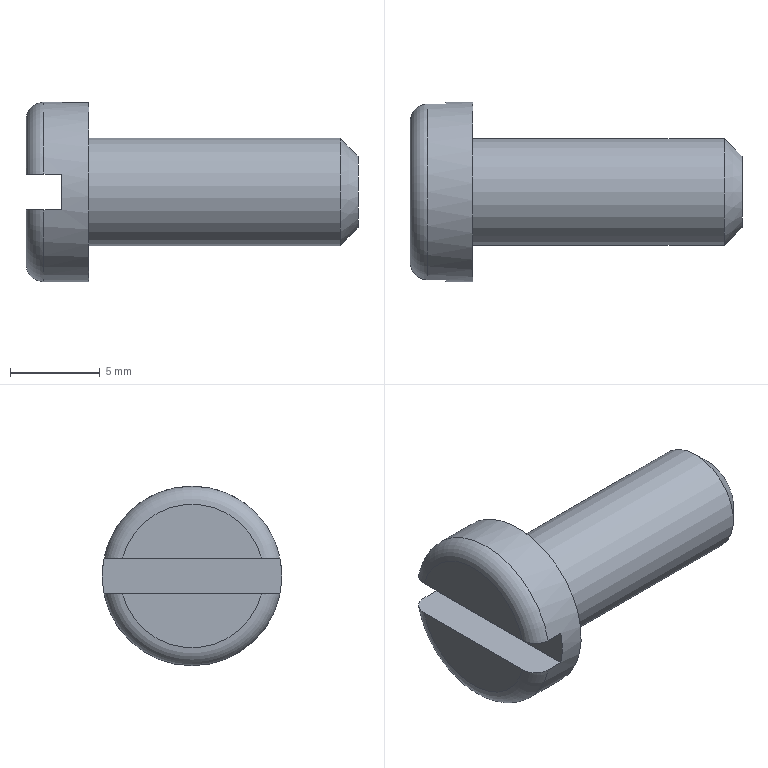Component | NX | SLOTTED_CAP_SCREW | 1 solid | 12 faces | box 18.5 x 10 x 10 mm | volume 645 mm3 | plane 7 | cylinder 2 | torus 2 | cone 1 | commonest cylinder face diameters 10 x1 6 x1
STEP:
#1=CARTESIAN_POINT('',(0.,0.,0.));
#2=DIRECTION('',(0.,0.,1.));
#3=DIRECTION('',(1.,0.,0.));
#4=AXIS2_PLACEMENT_3D('',#1,#2,#3);
#5=CARTESIAN_POINT('',(-33.6,-11.127,-0.5));
#6=VERTEX_POINT('',#5);
#7=CARTESIAN_POINT('',(-33.6,-18.873,-0.5));
#8=VERTEX_POINT('',#7);
#9=CARTESIAN_POINT('',(-33.6,11.305,-0.5));
#10=DIRECTION('',(0.,-1.,0.));
#11=VECTOR('',#10,1.);
#12=LINE('',#9,#11);
#13=CARTESIAN_POINT('',(-33.6,-15.,0.5));
#14=DIRECTION('',(-1.,0.,0.));
#15=DIRECTION('',(0.,0.,-1.));
#16=AXIS2_PLACEMENT_3D('',#13,#14,#15);
#17=PLANE('',#16);
#18=CARTESIAN_POINT('',(1.,-26.305));
#19=DIRECTION('',(0.,1.));
#20=VECTOR('',#19,1.);
#21=LINE('',#18,#20);
#22=(GEOMETRIC_REPRESENTATION_CONTEXT(2)PARAMETRIC_REPRESENTATION_CONTEXT()REPRESENTATION_CONTEXT('',''));
#23=DEFINITIONAL_REPRESENTATION('',(#21),#22);
#24=PCURVE('',#17,#23);
#25=CARTESIAN_POINT('',(-33.6,11.305,-0.5));
#26=DIRECTION('',(0.,0.,-1.));
#27=DIRECTION('',(1.,0.,0.));
#28=AXIS2_PLACEMENT_3D('',#25,#26,#27);
#29=PLANE('',#28);
#30=CARTESIAN_POINT('',(0.,0.));
#31=DIRECTION('',(0.,1.));
#32=VECTOR('',#31,1.);
#33=LINE('',#30,#32);
#34=(GEOMETRIC_REPRESENTATION_CONTEXT(2)PARAMETRIC_REPRESENTATION_CONTEXT()REPRESENTATION_CONTEXT('',''));
#35=DEFINITIONAL_REPRESENTATION('',(#33),#34);
#36=PCURVE('',#29,#35);
#37=SURFACE_CURVE('',#12,(#24,#36),.PCURVE_S1.);
#38=EDGE_CURVE('',#6,#8,#37,.T.);
#39=ORIENTED_EDGE('',*,*,#38,.F.);
#40=CARTESIAN_POINT('',(-33.6,-15.,0.5));
#41=DIRECTION('',(-1.,0.,0.));
#42=DIRECTION('',(0.,0.,-1.));
#43=AXIS2_PLACEMENT_3D('',#40,#41,#42);
#44=CIRCLE('',#43,4.);
#45=CARTESIAN_POINT('',(0.,0.));
#46=DIRECTION('',(1.,0.));
#47=AXIS2_PLACEMENT_2D('',#45,#46);
#48=CIRCLE('',#47,4.);
#49=(GEOMETRIC_REPRESENTATION_CONTEXT(2)PARAMETRIC_REPRESENTATION_CONTEXT()REPRESENTATION_CONTEXT('',''));
#50=DEFINITIONAL_REPRESENTATION('',(#48),#49);
#51=PCURVE('',#17,#50);
#52=CARTESIAN_POINT('',(-32.6,-15.,0.5));
#53=DIRECTION('',(-1.,0.,0.));
#54=DIRECTION('',(0.,0.,-1.));
#55=AXIS2_PLACEMENT_3D('',#52,#53,#54);
#56=TOROIDAL_SURFACE('',#55,4.,1.);
#57=CARTESIAN_POINT('',(0.,1.571));
#58=DIRECTION('',(1.,-0.));
#59=VECTOR('',#58,1.);
#60=LINE('',#57,#59);
#61=(GEOMETRIC_REPRESENTATION_CONTEXT(2)PARAMETRIC_REPRESENTATION_CONTEXT()REPRESENTATION_CONTEXT('',''));
#62=DEFINITIONAL_REPRESENTATION('',(#60),#61);
#63=PCURVE('',#56,#62);
#64=SURFACE_CURVE('',#44,(#51,#63),.PCURVE_S1.);
#65=EDGE_CURVE('',#6,#8,#64,.T.);
#66=ORIENTED_EDGE('',*,*,#65,.T.);
#67=EDGE_LOOP('',(#39,#66));
#68=FACE_BOUND('',#67,.T.);
#69=ADVANCED_FACE('',(#68),#17,.T.);
#70=CARTESIAN_POINT('',(-33.6,-11.127,1.5));
#71=VERTEX_POINT('',#70);
#72=CARTESIAN_POINT('',(-33.6,-18.873,1.5));
#73=VERTEX_POINT('',#72);
#74=CARTESIAN_POINT('',(-33.6,11.305,1.5));
#75=DIRECTION('',(0.,-1.,0.));
#76=VECTOR('',#75,1.);
#77=LINE('',#74,#76);
#78=CARTESIAN_POINT('',(-33.6,-15.,0.5));
#79=DIRECTION('',(-1.,0.,0.));
#80=DIRECTION('',(0.,0.,-1.));
#81=AXIS2_PLACEMENT_3D('',#78,#79,#80);
#82=PLANE('',#81);
#83=CARTESIAN_POINT('',(-1.,-26.305));
#84=DIRECTION('',(0.,1.));
#85=VECTOR('',#84,1.);
#86=LINE('',#83,#85);
#87=(GEOMETRIC_REPRESENTATION_CONTEXT(2)PARAMETRIC_REPRESENTATION_CONTEXT()REPRESENTATION_CONTEXT('',''));
#88=DEFINITIONAL_REPRESENTATION('',(#86),#87);
#89=PCURVE('',#82,#88);
#90=CARTESIAN_POINT('',(-33.6,-38.695,1.5));
#91=DIRECTION('',(0.,0.,1.));
#92=DIRECTION('',(-1.,0.,0.));
#93=AXIS2_PLACEMENT_3D('',#90,#91,#92);
#94=PLANE('',#93);
#95=CARTESIAN_POINT('',(0.,-50.));
#96=DIRECTION('',(0.,1.));
#97=VECTOR('',#96,1.);
#98=LINE('',#95,#97);
#99=(GEOMETRIC_REPRESENTATION_CONTEXT(2)PARAMETRIC_REPRESENTATION_CONTEXT()REPRESENTATION_CONTEXT('',''));
#100=DEFINITIONAL_REPRESENTATION('',(#98),#99);
#101=PCURVE('',#94,#100);
#102=SURFACE_CURVE('',#77,(#89,#101),.PCURVE_S1.);
#103=EDGE_CURVE('',#71,#73,#102,.T.);
#104=ORIENTED_EDGE('',*,*,#103,.T.);
#105=CARTESIAN_POINT('',(-33.6,-15.,0.5));
#106=DIRECTION('',(-1.,0.,0.));
#107=DIRECTION('',(0.,0.,-1.));
#108=AXIS2_PLACEMENT_3D('',#105,#106,#107);
#109=CIRCLE('',#108,4.);
#110=CARTESIAN_POINT('',(0.,0.));
#111=DIRECTION('',(1.,0.));
#112=AXIS2_PLACEMENT_2D('',#110,#111);
#113=CIRCLE('',#112,4.);
#114=(GEOMETRIC_REPRESENTATION_CONTEXT(2)PARAMETRIC_REPRESENTATION_CONTEXT()REPRESENTATION_CONTEXT('',''));
#115=DEFINITIONAL_REPRESENTATION('',(#113),#114);
#116=PCURVE('',#82,#115);
#117=CARTESIAN_POINT('',(-32.6,-15.,0.5));
#118=DIRECTION('',(-1.,0.,0.));
#119=DIRECTION('',(0.,0.,-1.));
#120=AXIS2_PLACEMENT_3D('',#117,#118,#119);
#121=TOROIDAL_SURFACE('',#120,4.,1.);
#122=CARTESIAN_POINT('',(0.,1.571));
#123=DIRECTION('',(1.,-0.));
#124=VECTOR('',#123,1.);
#125=LINE('',#122,#124);
#126=(GEOMETRIC_REPRESENTATION_CONTEXT(2)PARAMETRIC_REPRESENTATION_CONTEXT()REPRESENTATION_CONTEXT('',''));
#127=DEFINITIONAL_REPRESENTATION('',(#125),#126);
#128=PCURVE('',#121,#127);
#129=SURFACE_CURVE('',#109,(#116,#128),.PCURVE_S1.);
#130=EDGE_CURVE('',#73,#71,#129,.T.);
#131=ORIENTED_EDGE('',*,*,#130,.T.);
#132=EDGE_LOOP('',(#104,#131));
#133=FACE_BOUND('',#132,.T.);
#134=ADVANCED_FACE('',(#133),#82,.T.);
#135=CARTESIAN_POINT('',(-30.1,-15.,3.5));
#136=VERTEX_POINT('',#135);
#137=CARTESIAN_POINT('',(-30.1,-15.,0.5));
#138=DIRECTION('',(1.,0.,0.));
#139=DIRECTION('',(0.,0.,1.));
#140=AXIS2_PLACEMENT_3D('',#137,#138,#139);
#141=CIRCLE('',#140,3.);
#142=CARTESIAN_POINT('',(-30.1,-15.,0.5));
#143=DIRECTION('',(1.,0.,0.));
#144=DIRECTION('',(0.,0.,1.));
#145=AXIS2_PLACEMENT_3D('',#142,#143,#144);
#146=PLANE('',#145);
#147=CARTESIAN_POINT('',(-0.,0.));
#148=DIRECTION('',(1.,0.));
#149=AXIS2_PLACEMENT_2D('',#147,#148);
#150=CIRCLE('',#149,3.);
#151=(GEOMETRIC_REPRESENTATION_CONTEXT(2)PARAMETRIC_REPRESENTATION_CONTEXT()REPRESENTATION_CONTEXT('',''));
#152=DEFINITIONAL_REPRESENTATION('',(#150),#151);
#153=PCURVE('',#146,#152);
#154=CARTESIAN_POINT('',(-30.1,-15.,0.5));
#155=DIRECTION('',(1.,0.,0.));
#156=DIRECTION('',(0.,0.,1.));
#157=AXIS2_PLACEMENT_3D('',#154,#155,#156);
#158=CYLINDRICAL_SURFACE('',#157,3.);
#159=CARTESIAN_POINT('',(0.,0.));
#160=DIRECTION('',(1.,0.));
#161=VECTOR('',#160,1.);
#162=LINE('',#159,#161);
#163=(GEOMETRIC_REPRESENTATION_CONTEXT(2)PARAMETRIC_REPRESENTATION_CONTEXT()REPRESENTATION_CONTEXT('',''));
#164=DEFINITIONAL_REPRESENTATION('',(#162),#163);
#165=PCURVE('',#158,#164);
#166=SURFACE_CURVE('',#141,(#153,#165),.PCURVE_S1.);
#167=EDGE_CURVE('',#136,#136,#166,.T.);
#168=ORIENTED_EDGE('',*,*,#167,.F.);
#169=EDGE_LOOP('',(#168));
#170=FACE_BOUND('',#169,.T.);
#171=CARTESIAN_POINT('',(-30.1,-15.,-4.5));
#172=VERTEX_POINT('',#171);
#173=CARTESIAN_POINT('',(-30.1,-15.,0.5));
#174=DIRECTION('',(-1.,0.,0.));
#175=DIRECTION('',(0.,0.,-1.));
#176=AXIS2_PLACEMENT_3D('',#173,#174,#175);
#177=CIRCLE('',#176,5.);
#178=CARTESIAN_POINT('',(-5.,0.));
#179=CARTESIAN_POINT('',(-5.,8.66));
#180=CARTESIAN_POINT('',(2.5,4.33));
#181=CARTESIAN_POINT('',(10.,0.));
#182=CARTESIAN_POINT('',(2.5,-4.33));
#183=CARTESIAN_POINT('',(-5.,-8.66));
#184=CARTESIAN_POINT('',(-5.,0.));
#185=(BOUNDED_CURVE()B_SPLINE_CURVE(2,(#178,#179,#180,#181,#182,#183,#184),.UNSPECIFIED.,.T.,.F.)B_SPLINE_CURVE_WITH_KNOTS((1,2,2,2,2,1),(-2.094,0.,2.094,4.189,6.283,8.378),.UNSPECIFIED.)CURVE()GEOMETRIC_REPRESENTATION_ITEM()RATIONAL_B_SPLINE_CURVE((1.,0.5,1.,0.5,1.,0.5,1.))REPRESENTATION_ITEM(''));
#186=(GEOMETRIC_REPRESENTATION_CONTEXT(2)PARAMETRIC_REPRESENTATION_CONTEXT()REPRESENTATION_CONTEXT('',''));
#187=DEFINITIONAL_REPRESENTATION('',(#185),#186);
#188=PCURVE('',#146,#187);
#189=CARTESIAN_POINT('',(-30.1,-15.,0.5));
#190=DIRECTION('',(-1.,0.,0.));
#191=DIRECTION('',(0.,0.,-1.));
#192=AXIS2_PLACEMENT_3D('',#189,#190,#191);
#193=CYLINDRICAL_SURFACE('',#192,5.);
#194=CARTESIAN_POINT('',(0.,0.));
#195=DIRECTION('',(1.,0.));
#196=VECTOR('',#195,1.);
#197=LINE('',#194,#196);
#198=(GEOMETRIC_REPRESENTATION_CONTEXT(2)PARAMETRIC_REPRESENTATION_CONTEXT()REPRESENTATION_CONTEXT('',''));
#199=DEFINITIONAL_REPRESENTATION('',(#197),#198);
#200=PCURVE('',#193,#199);
#201=SURFACE_CURVE('',#177,(#188,#200),.PCURVE_S1.);
#202=EDGE_CURVE('',#172,#172,#201,.T.);
#203=ORIENTED_EDGE('',*,*,#202,.F.);
#204=EDGE_LOOP('',(#203));
#205=FACE_BOUND('',#204,.T.);
#206=ADVANCED_FACE('',(#170,#205),#146,.T.);
#207=CARTESIAN_POINT('',(-32.6,-19.899,-0.5));
#208=VERTEX_POINT('',#207);
#209=CARTESIAN_POINT('',(-31.6,-19.899,-0.5));
#210=VERTEX_POINT('',#209);
#211=CARTESIAN_POINT('',(-30.1,-19.899,-0.5));
#212=DIRECTION('',(1.,0.,0.));
#213=VECTOR('',#212,1.);
#214=LINE('',#211,#213);
#215=CARTESIAN_POINT('',(1.369,0.));
#216=DIRECTION('',(0.,-1.));
#217=VECTOR('',#216,1.);
#218=LINE('',#215,#217);
#219=(GEOMETRIC_REPRESENTATION_CONTEXT(2)PARAMETRIC_REPRESENTATION_CONTEXT()REPRESENTATION_CONTEXT('',''));
#220=DEFINITIONAL_REPRESENTATION('',(#218),#219);
#221=PCURVE('',#193,#220);
#222=CARTESIAN_POINT('',(3.5,31.204));
#223=DIRECTION('',(1.,0.));
#224=VECTOR('',#223,1.);
#225=LINE('',#222,#224);
#226=(GEOMETRIC_REPRESENTATION_CONTEXT(2)PARAMETRIC_REPRESENTATION_CONTEXT()REPRESENTATION_CONTEXT('',''));
#227=DEFINITIONAL_REPRESENTATION('',(#225),#226);
#228=PCURVE('',#29,#227);
#229=SURFACE_CURVE('',#214,(#221,#228),.PCURVE_S1.);
#230=EDGE_CURVE('',#208,#210,#229,.T.);
#231=ORIENTED_EDGE('',*,*,#230,.F.);
#232=CARTESIAN_POINT('',(-32.6,-15.,-4.5));
#233=VERTEX_POINT('',#232);
#234=CARTESIAN_POINT('',(-32.6,-15.,0.5));
#235=DIRECTION('',(1.,0.,0.));
#236=DIRECTION('',(0.,0.,-1.));
#237=AXIS2_PLACEMENT_3D('',#234,#235,#236);
#238=CIRCLE('',#237,5.);
#239=CARTESIAN_POINT('',(6.283,2.5));
#240=DIRECTION('',(-1.,0.));
#241=VECTOR('',#240,1.);
#242=LINE('',#239,#241);
#243=(GEOMETRIC_REPRESENTATION_CONTEXT(2)PARAMETRIC_REPRESENTATION_CONTEXT()REPRESENTATION_CONTEXT('',''));
#244=DEFINITIONAL_REPRESENTATION('',(#242),#243);
#245=PCURVE('',#193,#244);
#246=CARTESIAN_POINT('',(12.566,0.));
#247=DIRECTION('',(-1.,0.));
#248=VECTOR('',#247,1.);
#249=LINE('',#246,#248);
#250=(GEOMETRIC_REPRESENTATION_CONTEXT(2)PARAMETRIC_REPRESENTATION_CONTEXT()REPRESENTATION_CONTEXT('',''));
#251=DEFINITIONAL_REPRESENTATION('',(#249),#250);
#252=PCURVE('',#56,#251);
#253=SURFACE_CURVE('',#238,(#245,#252),.PCURVE_S1.);
#254=EDGE_CURVE('',#208,#233,#253,.T.);
#255=ORIENTED_EDGE('',*,*,#254,.T.);
#256=CARTESIAN_POINT('',(-30.1,-15.,-4.5));
#257=CARTESIAN_POINT('',(-32.6,-15.,-4.5));
#258=B_SPLINE_CURVE_WITH_KNOTS('',1,(#256,#257),.UNSPECIFIED.,.F.,.F.,(2,2),(0.,2.5),.PIECEWISE_BEZIER_KNOTS.);
#259=CARTESIAN_POINT('',(0.,0.));
#260=DIRECTION('',(0.,1.));
#261=VECTOR('',#260,1.);
#262=LINE('',#259,#261);
#263=(GEOMETRIC_REPRESENTATION_CONTEXT(2)PARAMETRIC_REPRESENTATION_CONTEXT()REPRESENTATION_CONTEXT('',''));
#264=DEFINITIONAL_REPRESENTATION('',(#262),#263);
#265=PCURVE('',#193,#264);
#266=CARTESIAN_POINT('',(6.283,0.));
#267=DIRECTION('',(0.,1.));
#268=VECTOR('',#267,1.);
#269=LINE('',#266,#268);
#270=(GEOMETRIC_REPRESENTATION_CONTEXT(2)PARAMETRIC_REPRESENTATION_CONTEXT()REPRESENTATION_CONTEXT('',''));
#271=DEFINITIONAL_REPRESENTATION('',(#269),#270);
#272=PCURVE('',#193,#271);
#273=SEAM_CURVE('',#258,(#265,#272),.PCURVE_S1.);
#274=EDGE_CURVE('',#172,#233,#273,.T.);
#275=ORIENTED_EDGE('',*,*,#274,.F.);
#276=ORIENTED_EDGE('',*,*,#202,.T.);
#277=ORIENTED_EDGE('',*,*,#274,.T.);
#278=CARTESIAN_POINT('',(-32.6,-10.101,-0.5));
#279=VERTEX_POINT('',#278);
#280=CARTESIAN_POINT('',(-32.6,-15.,0.5));
#281=DIRECTION('',(1.,0.,0.));
#282=DIRECTION('',(0.,0.,-1.));
#283=AXIS2_PLACEMENT_3D('',#280,#281,#282);
#284=CIRCLE('',#283,5.);
#285=CARTESIAN_POINT('',(12.566,2.5));
#286=DIRECTION('',(-1.,0.));
#287=VECTOR('',#286,1.);
#288=LINE('',#285,#287);
#289=(GEOMETRIC_REPRESENTATION_CONTEXT(2)PARAMETRIC_REPRESENTATION_CONTEXT()REPRESENTATION_CONTEXT('',''));
#290=DEFINITIONAL_REPRESENTATION('',(#288),#289);
#291=PCURVE('',#193,#290);
#292=CARTESIAN_POINT('',(12.566,0.));
#293=DIRECTION('',(-1.,0.));
#294=VECTOR('',#293,1.);
#295=LINE('',#292,#294);
#296=(GEOMETRIC_REPRESENTATION_CONTEXT(2)PARAMETRIC_REPRESENTATION_CONTEXT()REPRESENTATION_CONTEXT('',''));
#297=DEFINITIONAL_REPRESENTATION('',(#295),#296);
#298=PCURVE('',#56,#297);
#299=SURFACE_CURVE('',#284,(#291,#298),.PCURVE_S1.);
#300=EDGE_CURVE('',#233,#279,#299,.T.);
#301=ORIENTED_EDGE('',*,*,#300,.T.);
#302=CARTESIAN_POINT('',(-31.6,-10.101,-0.5));
#303=VERTEX_POINT('',#302);
#304=CARTESIAN_POINT('',(-30.1,-10.101,-0.5));
#305=DIRECTION('',(-1.,0.,0.));
#306=VECTOR('',#305,1.);
#307=LINE('',#304,#306);
#308=CARTESIAN_POINT('',(4.914,0.));
#309=DIRECTION('',(0.,1.));
#310=VECTOR('',#309,1.);
#311=LINE('',#308,#310);
#312=(GEOMETRIC_REPRESENTATION_CONTEXT(2)PARAMETRIC_REPRESENTATION_CONTEXT()REPRESENTATION_CONTEXT('',''));
#313=DEFINITIONAL_REPRESENTATION('',(#311),#312);
#314=PCURVE('',#193,#313);
#315=CARTESIAN_POINT('',(3.5,21.406));
#316=DIRECTION('',(-1.,0.));
#317=VECTOR('',#316,1.);
#318=LINE('',#315,#317);
#319=(GEOMETRIC_REPRESENTATION_CONTEXT(2)PARAMETRIC_REPRESENTATION_CONTEXT()REPRESENTATION_CONTEXT('',''));
#320=DEFINITIONAL_REPRESENTATION('',(#318),#319);
#321=PCURVE('',#29,#320);
#322=SURFACE_CURVE('',#307,(#314,#321),.PCURVE_S1.);
#323=EDGE_CURVE('',#303,#279,#322,.T.);
#324=ORIENTED_EDGE('',*,*,#323,.F.);
#325=CARTESIAN_POINT('',(-31.6,-10.101,1.5));
#326=VERTEX_POINT('',#325);
#327=CARTESIAN_POINT('',(-31.6,-15.,0.5));
#328=DIRECTION('',(-1.,0.,0.));
#329=DIRECTION('',(0.,0.,1.));
#330=AXIS2_PLACEMENT_3D('',#327,#328,#329);
#331=CIRCLE('',#330,5.);
#332=CARTESIAN_POINT('',(3.142,1.5));
#333=DIRECTION('',(1.,0.));
#334=VECTOR('',#333,1.);
#335=LINE('',#332,#334);
#336=(GEOMETRIC_REPRESENTATION_CONTEXT(2)PARAMETRIC_REPRESENTATION_CONTEXT()REPRESENTATION_CONTEXT('',''));
#337=DEFINITIONAL_REPRESENTATION('',(#335),#336);
#338=PCURVE('',#193,#337);
#339=CARTESIAN_POINT('',(-31.6,11.305,1.5));
#340=DIRECTION('',(1.,0.,0.));
#341=DIRECTION('',(0.,0.,1.));
#342=AXIS2_PLACEMENT_3D('',#339,#340,#341);
#343=PLANE('',#342);
#344=CARTESIAN_POINT('',(4.,26.305));
#345=CARTESIAN_POINT('',(4.,17.645));
#346=CARTESIAN_POINT('',(-3.5,21.975));
#347=CARTESIAN_POINT('',(-11.,26.305));
#348=CARTESIAN_POINT('',(-3.5,30.636));
#349=CARTESIAN_POINT('',(4.,34.966));
#350=CARTESIAN_POINT('',(4.,26.305));
#351=(BOUNDED_CURVE()B_SPLINE_CURVE(2,(#344,#345,#346,#347,#348,#349,#350),.UNSPECIFIED.,.T.,.F.)B_SPLINE_CURVE_WITH_KNOTS((1,2,2,2,2,1),(-2.094,0.,2.094,4.189,6.283,8.378),.UNSPECIFIED.)CURVE()GEOMETRIC_REPRESENTATION_ITEM()RATIONAL_B_SPLINE_CURVE((1.,0.5,1.,0.5,1.,0.5,1.))REPRESENTATION_ITEM(''));
#352=(GEOMETRIC_REPRESENTATION_CONTEXT(2)PARAMETRIC_REPRESENTATION_CONTEXT()REPRESENTATION_CONTEXT('',''));
#353=DEFINITIONAL_REPRESENTATION('',(#351),#352);
#354=PCURVE('',#343,#353);
#355=SURFACE_CURVE('',#331,(#338,#354),.PCURVE_S1.);
#356=EDGE_CURVE('',#326,#303,#355,.T.);
#357=ORIENTED_EDGE('',*,*,#356,.F.);
#358=CARTESIAN_POINT('',(-32.6,-10.101,1.5));
#359=VERTEX_POINT('',#358);
#360=CARTESIAN_POINT('',(-30.1,-10.101,1.5));
#361=DIRECTION('',(1.,0.,0.));
#362=VECTOR('',#361,1.);
#363=LINE('',#360,#362);
#364=CARTESIAN_POINT('',(4.511,0.));
#365=DIRECTION('',(0.,-1.));
#366=VECTOR('',#365,1.);
#367=LINE('',#364,#366);
#368=(GEOMETRIC_REPRESENTATION_CONTEXT(2)PARAMETRIC_REPRESENTATION_CONTEXT()REPRESENTATION_CONTEXT('',''));
#369=DEFINITIONAL_REPRESENTATION('',(#367),#368);
#370=PCURVE('',#193,#369);
#371=CARTESIAN_POINT('',(-3.5,-28.594));
#372=DIRECTION('',(-1.,0.));
#373=VECTOR('',#372,1.);
#374=LINE('',#371,#373);
#375=(GEOMETRIC_REPRESENTATION_CONTEXT(2)PARAMETRIC_REPRESENTATION_CONTEXT()REPRESENTATION_CONTEXT('',''));
#376=DEFINITIONAL_REPRESENTATION('',(#374),#375);
#377=PCURVE('',#94,#376);
#378=SURFACE_CURVE('',#363,(#370,#377),.PCURVE_S1.);
#379=EDGE_CURVE('',#359,#326,#378,.T.);
#380=ORIENTED_EDGE('',*,*,#379,.F.);
#381=CARTESIAN_POINT('',(-32.6,-19.899,1.5));
#382=VERTEX_POINT('',#381);
#383=CARTESIAN_POINT('',(-32.6,-15.,0.5));
#384=DIRECTION('',(1.,0.,0.));
#385=DIRECTION('',(0.,0.,-1.));
#386=AXIS2_PLACEMENT_3D('',#383,#384,#385);
#387=CIRCLE('',#386,5.);
#388=CARTESIAN_POINT('',(6.283,2.5));
#389=DIRECTION('',(-1.,0.));
#390=VECTOR('',#389,1.);
#391=LINE('',#388,#390);
#392=(GEOMETRIC_REPRESENTATION_CONTEXT(2)PARAMETRIC_REPRESENTATION_CONTEXT()REPRESENTATION_CONTEXT('',''));
#393=DEFINITIONAL_REPRESENTATION('',(#391),#392);
#394=PCURVE('',#193,#393);
#395=CARTESIAN_POINT('',(6.283,0.));
#396=DIRECTION('',(-1.,0.));
#397=VECTOR('',#396,1.);
#398=LINE('',#395,#397);
#399=(GEOMETRIC_REPRESENTATION_CONTEXT(2)PARAMETRIC_REPRESENTATION_CONTEXT()REPRESENTATION_CONTEXT('',''));
#400=DEFINITIONAL_REPRESENTATION('',(#398),#399);
#401=PCURVE('',#121,#400);
#402=SURFACE_CURVE('',#387,(#394,#401),.PCURVE_S1.);
#403=EDGE_CURVE('',#359,#382,#402,.T.);
#404=ORIENTED_EDGE('',*,*,#403,.T.);
#405=CARTESIAN_POINT('',(-31.6,-19.899,1.5));
#406=VERTEX_POINT('',#405);
#407=CARTESIAN_POINT('',(-30.1,-19.899,1.5));
#408=DIRECTION('',(-1.,0.,0.));
#409=VECTOR('',#408,1.);
#410=LINE('',#407,#409);
#411=CARTESIAN_POINT('',(1.772,0.));
#412=DIRECTION('',(0.,1.));
#413=VECTOR('',#412,1.);
#414=LINE('',#411,#413);
#415=(GEOMETRIC_REPRESENTATION_CONTEXT(2)PARAMETRIC_REPRESENTATION_CONTEXT()REPRESENTATION_CONTEXT('',''));
#416=DEFINITIONAL_REPRESENTATION('',(#414),#415);
#417=PCURVE('',#193,#416);
#418=CARTESIAN_POINT('',(-3.5,-18.796));
#419=DIRECTION('',(1.,0.));
#420=VECTOR('',#419,1.);
#421=LINE('',#418,#420);
#422=(GEOMETRIC_REPRESENTATION_CONTEXT(2)PARAMETRIC_REPRESENTATION_CONTEXT()REPRESENTATION_CONTEXT('',''));
#423=DEFINITIONAL_REPRESENTATION('',(#421),#422);
#424=PCURVE('',#94,#423);
#425=SURFACE_CURVE('',#410,(#417,#424),.PCURVE_S1.);
#426=EDGE_CURVE('',#406,#382,#425,.T.);
#427=ORIENTED_EDGE('',*,*,#426,.F.);
#428=CARTESIAN_POINT('',(-31.6,-15.,0.5));
#429=DIRECTION('',(-1.,0.,0.));
#430=DIRECTION('',(0.,0.,1.));
#431=AXIS2_PLACEMENT_3D('',#428,#429,#430);
#432=CIRCLE('',#431,5.);
#433=CARTESIAN_POINT('',(-3.142,1.5));
#434=DIRECTION('',(1.,0.));
#435=VECTOR('',#434,1.);
#436=LINE('',#433,#435);
#437=(GEOMETRIC_REPRESENTATION_CONTEXT(2)PARAMETRIC_REPRESENTATION_CONTEXT()REPRESENTATION_CONTEXT('',''));
#438=DEFINITIONAL_REPRESENTATION('',(#436),#437);
#439=PCURVE('',#193,#438);
#440=CARTESIAN_POINT('',(4.,26.305));
#441=CARTESIAN_POINT('',(4.,17.645));
#442=CARTESIAN_POINT('',(-3.5,21.975));
#443=CARTESIAN_POINT('',(-11.,26.305));
#444=CARTESIAN_POINT('',(-3.5,30.636));
#445=CARTESIAN_POINT('',(4.,34.966));
#446=CARTESIAN_POINT('',(4.,26.305));
#447=(BOUNDED_CURVE()B_SPLINE_CURVE(2,(#440,#441,#442,#443,#444,#445,#446),.UNSPECIFIED.,.T.,.F.)B_SPLINE_CURVE_WITH_KNOTS((1,2,2,2,2,1),(-2.094,0.,2.094,4.189,6.283,8.378),.UNSPECIFIED.)CURVE()GEOMETRIC_REPRESENTATION_ITEM()RATIONAL_B_SPLINE_CURVE((1.,0.5,1.,0.5,1.,0.5,1.))REPRESENTATION_ITEM(''));
#448=(GEOMETRIC_REPRESENTATION_CONTEXT(2)PARAMETRIC_REPRESENTATION_CONTEXT()REPRESENTATION_CONTEXT('',''));
#449=DEFINITIONAL_REPRESENTATION('',(#447),#448);
#450=PCURVE('',#343,#449);
#451=SURFACE_CURVE('',#432,(#439,#450),.PCURVE_S1.);
#452=EDGE_CURVE('',#210,#406,#451,.T.);
#453=ORIENTED_EDGE('',*,*,#452,.F.);
#454=EDGE_LOOP('',(#231,#255,#275,#276,#277,#301,#324,#357,#380,#404,#427,#453));
#455=FACE_BOUND('',#454,.T.);
#456=ADVANCED_FACE('',(#455),#193,.T.);
#457=ORIENTED_EDGE('',*,*,#323,.T.);
#458=CARTESIAN_POINT('',(-32.6,-10.101,-0.5));
#459=CARTESIAN_POINT('',(-32.71,-10.101,-0.5));
#460=CARTESIAN_POINT('',(-32.822,-10.12,-0.5));
#461=CARTESIAN_POINT('',(-32.926,-10.157,-0.5));
#462=CARTESIAN_POINT('',(-33.03,-10.193,-0.5));
#463=CARTESIAN_POINT('',(-33.129,-10.248,-0.5));
#464=CARTESIAN_POINT('',(-33.215,-10.317,-0.5));
#465=CARTESIAN_POINT('',(-33.301,-10.386,-0.5));
#466=CARTESIAN_POINT('',(-33.378,-10.471,-0.5));
#467=CARTESIAN_POINT('',(-33.437,-10.564,-0.5));
#468=CARTESIAN_POINT('',(-33.498,-10.66,-0.5));
#469=CARTESIAN_POINT('',(-33.543,-10.767,-0.5));
#470=CARTESIAN_POINT('',(-33.57,-10.877,-0.5));
#471=CARTESIAN_POINT('',(-33.59,-10.958,-0.5));
#472=CARTESIAN_POINT('',(-33.6,-11.043,-0.5));
#473=CARTESIAN_POINT('',(-33.6,-11.127,-0.5));
#474=B_SPLINE_CURVE_WITH_KNOTS('',3,(#458,#459,#460,#461,#462,#463,#464,#465,#466,#467,#468,#469,#470,#471,#472,#473),.UNSPECIFIED.,.F.,.F.,(4,3,3,3,3,4),(0.,0.2087,0.4173,0.6275,0.8418,1.),.UNSPECIFIED.);
#475=CARTESIAN_POINT('',(1.,21.406));
#476=CARTESIAN_POINT('',(0.8899,21.406));
#477=CARTESIAN_POINT('',(0.7782,21.426));
#478=CARTESIAN_POINT('',(0.6743,21.462));
#479=CARTESIAN_POINT('',(0.5704,21.499));
#480=CARTESIAN_POINT('',(0.4714,21.554));
#481=CARTESIAN_POINT('',(0.3853,21.622));
#482=CARTESIAN_POINT('',(0.2985,21.691));
#483=CARTESIAN_POINT('',(0.2224,21.776));
#484=CARTESIAN_POINT('',(0.1628,21.87));
#485=CARTESIAN_POINT('',(0.102,21.965));
#486=CARTESIAN_POINT('',(0.05666,22.072));
#487=CARTESIAN_POINT('',(0.02992,22.182));
#488=CARTESIAN_POINT('',(0.01006,22.264));
#489=CARTESIAN_POINT('',(0.,22.348));
#490=CARTESIAN_POINT('',(0.,22.432));
#491=B_SPLINE_CURVE_WITH_KNOTS('',3,(#475,#476,#477,#478,#479,#480,#481,#482,#483,#484,#485,#486,#487,#488,#489,#490),.UNSPECIFIED.,.F.,.F.,(4,3,3,3,3,4),(0.,0.2087,0.4173,0.6275,0.8418,1.),.UNSPECIFIED.);
#492=(GEOMETRIC_REPRESENTATION_CONTEXT(2)PARAMETRIC_REPRESENTATION_CONTEXT()REPRESENTATION_CONTEXT('',''));
#493=DEFINITIONAL_REPRESENTATION('',(#491),#492);
#494=PCURVE('',#29,#493);
#495=CARTESIAN_POINT('',(4.914,0.));
#496=CARTESIAN_POINT('',(4.914,0.02399));
#497=CARTESIAN_POINT('',(4.914,0.07211));
#498=CARTESIAN_POINT('',(4.914,0.1445));
#499=CARTESIAN_POINT('',(4.915,0.217));
#500=CARTESIAN_POINT('',(4.915,0.2893));
#501=CARTESIAN_POINT('',(4.916,0.3611));
#502=CARTESIAN_POINT('',(4.918,0.4332));
#503=CARTESIAN_POINT('',(4.919,0.5053));
#504=CARTESIAN_POINT('',(4.921,0.5774));
#505=CARTESIAN_POINT('',(4.922,0.6491));
#506=CARTESIAN_POINT('',(4.924,0.7205));
#507=CARTESIAN_POINT('',(4.927,0.7921));
#508=CARTESIAN_POINT('',(4.929,0.8637));
#509=CARTESIAN_POINT('',(4.932,0.9351));
#510=CARTESIAN_POINT('',(4.935,1.006));
#511=CARTESIAN_POINT('',(4.938,1.077));
#512=CARTESIAN_POINT('',(4.941,1.148));
#513=CARTESIAN_POINT('',(4.945,1.219));
#514=CARTESIAN_POINT('',(4.948,1.289));
#515=CARTESIAN_POINT('',(4.952,1.359));
#516=CARTESIAN_POINT('',(4.956,1.43));
#517=CARTESIAN_POINT('',(4.961,1.501));
#518=CARTESIAN_POINT('',(4.964,1.547));
#519=CARTESIAN_POINT('',(4.965,1.571));
#520=B_SPLINE_CURVE_WITH_KNOTS('',3,(#495,#496,#497,#498,#499,#500,#501,#502,#503,#504,#505,#506,#507,#508,#509,#510,#511,#512,#513,#514,#515,#516,#517,#518,#519),.UNSPECIFIED.,.F.,.F.,(4,1,1,1,1,1,1,1,1,1,1,1,1,1,1,1,1,1,1,1,1,1,4),(0.,0.04545,0.09091,0.1364,0.1818,0.2273,0.2727,0.3182,0.3636,0.4091,0.4545,0.5,0.5455,0.5909,0.6364,0.6818,0.7273,0.7727,0.8182,0.8636,0.9091,0.9545,1.),.QUASI_UNIFORM_KNOTS.);
#521=(GEOMETRIC_REPRESENTATION_CONTEXT(2)PARAMETRIC_REPRESENTATION_CONTEXT()REPRESENTATION_CONTEXT('',''));
#522=DEFINITIONAL_REPRESENTATION('',(#520),#521);
#523=PCURVE('',#56,#522);
#524=SURFACE_CURVE('',#474,(#494,#523),.PCURVE_S1.);
#525=EDGE_CURVE('',#279,#6,#524,.T.);
#526=ORIENTED_EDGE('',*,*,#525,.T.);
#527=ORIENTED_EDGE('',*,*,#38,.T.);
#528=CARTESIAN_POINT('',(-33.6,-18.873,-0.5));
#529=CARTESIAN_POINT('',(-33.6,-18.99,-0.5));
#530=CARTESIAN_POINT('',(-33.58,-19.109,-0.5));
#531=CARTESIAN_POINT('',(-33.541,-19.22,-0.5));
#532=CARTESIAN_POINT('',(-33.503,-19.331,-0.5));
#533=CARTESIAN_POINT('',(-33.444,-19.437,-0.5));
#534=CARTESIAN_POINT('',(-33.37,-19.529,-0.5));
#535=CARTESIAN_POINT('',(-33.298,-19.618,-0.5));
#536=CARTESIAN_POINT('',(-33.209,-19.696,-0.5));
#537=CARTESIAN_POINT('',(-33.11,-19.756,-0.5));
#538=CARTESIAN_POINT('',(-33.014,-19.814,-0.5));
#539=CARTESIAN_POINT('',(-32.906,-19.857,-0.5));
#540=CARTESIAN_POINT('',(-32.796,-19.879,-0.5));
#541=CARTESIAN_POINT('',(-32.732,-19.892,-0.5));
#542=CARTESIAN_POINT('',(-32.666,-19.899,-0.5));
#543=CARTESIAN_POINT('',(-32.6,-19.899,-0.5));
#544=B_SPLINE_CURVE_WITH_KNOTS('',3,(#528,#529,#530,#531,#532,#533,#534,#535,#536,#537,#538,#539,#540,#541,#542,#543),.UNSPECIFIED.,.F.,.F.,(4,3,3,3,3,4),(0.,0.2225,0.4453,0.6637,0.8767,1.),.UNSPECIFIED.);
#545=CARTESIAN_POINT('',(0.,30.178));
#546=CARTESIAN_POINT('',(0.,30.296));
#547=CARTESIAN_POINT('',(0.01992,30.415));
#548=CARTESIAN_POINT('',(0.05857,30.526));
#549=CARTESIAN_POINT('',(0.09725,30.637));
#550=CARTESIAN_POINT('',(0.1558,30.743));
#551=CARTESIAN_POINT('',(0.2297,30.834));
#552=CARTESIAN_POINT('',(0.3021,30.924));
#553=CARTESIAN_POINT('',(0.3914,31.002));
#554=CARTESIAN_POINT('',(0.4899,31.062));
#555=CARTESIAN_POINT('',(0.586,31.12));
#556=CARTESIAN_POINT('',(0.6937,31.162));
#557=CARTESIAN_POINT('',(0.8038,31.185));
#558=CARTESIAN_POINT('',(0.8682,31.198));
#559=CARTESIAN_POINT('',(0.9343,31.204));
#560=CARTESIAN_POINT('',(1.,31.204));
#561=B_SPLINE_CURVE_WITH_KNOTS('',3,(#545,#546,#547,#548,#549,#550,#551,#552,#553,#554,#555,#556,#557,#558,#559,#560),.UNSPECIFIED.,.F.,.F.,(4,3,3,3,3,4),(0.,0.2225,0.4453,0.6637,0.8767,1.),.UNSPECIFIED.);
#562=(GEOMETRIC_REPRESENTATION_CONTEXT(2)PARAMETRIC_REPRESENTATION_CONTEXT()REPRESENTATION_CONTEXT('',''));
#563=DEFINITIONAL_REPRESENTATION('',(#561),#562);
#564=PCURVE('',#29,#563);
#565=CARTESIAN_POINT('',(7.601,1.571));
#566=CARTESIAN_POINT('',(7.603,1.548));
#567=CARTESIAN_POINT('',(7.606,1.501));
#568=CARTESIAN_POINT('',(7.61,1.431));
#569=CARTESIAN_POINT('',(7.614,1.36));
#570=CARTESIAN_POINT('',(7.618,1.29));
#571=CARTESIAN_POINT('',(7.622,1.22));
#572=CARTESIAN_POINT('',(7.625,1.149));
#573=CARTESIAN_POINT('',(7.629,1.078));
#574=CARTESIAN_POINT('',(7.632,1.007));
#575=CARTESIAN_POINT('',(7.635,0.9358));
#576=CARTESIAN_POINT('',(7.637,0.8649));
#577=CARTESIAN_POINT('',(7.64,0.7937));
#578=CARTESIAN_POINT('',(7.642,0.722));
#579=CARTESIAN_POINT('',(7.644,0.6501));
#580=CARTESIAN_POINT('',(7.646,0.5783));
#581=CARTESIAN_POINT('',(7.647,0.5068));
#582=CARTESIAN_POINT('',(7.649,0.4348));
#583=CARTESIAN_POINT('',(7.65,0.3626));
#584=CARTESIAN_POINT('',(7.651,0.2902));
#585=CARTESIAN_POINT('',(7.652,0.2182));
#586=CARTESIAN_POINT('',(7.652,0.1457));
#587=CARTESIAN_POINT('',(7.653,0.07276));
#588=CARTESIAN_POINT('',(7.653,0.0242));
#589=CARTESIAN_POINT('',(7.653,0.));
#590=B_SPLINE_CURVE_WITH_KNOTS('',3,(#565,#566,#567,#568,#569,#570,#571,#572,#573,#574,#575,#576,#577,#578,#579,#580,#581,#582,#583,#584,#585,#586,#587,#588,#589),.UNSPECIFIED.,.F.,.F.,(4,1,1,1,1,1,1,1,1,1,1,1,1,1,1,1,1,1,1,1,1,1,4),(0.,0.04545,0.09091,0.1364,0.1818,0.2273,0.2727,0.3182,0.3636,0.4091,0.4545,0.5,0.5455,0.5909,0.6364,0.6818,0.7273,0.7727,0.8182,0.8636,0.9091,0.9545,1.),.QUASI_UNIFORM_KNOTS.);
#591=(GEOMETRIC_REPRESENTATION_CONTEXT(2)PARAMETRIC_REPRESENTATION_CONTEXT()REPRESENTATION_CONTEXT('',''));
#592=DEFINITIONAL_REPRESENTATION('',(#590),#591);
#593=PCURVE('',#56,#592);
#594=SURFACE_CURVE('',#544,(#564,#593),.PCURVE_S1.);
#595=EDGE_CURVE('',#8,#208,#594,.T.);
#596=ORIENTED_EDGE('',*,*,#595,.T.);
#597=ORIENTED_EDGE('',*,*,#230,.T.);
#598=CARTESIAN_POINT('',(-31.6,11.305,-0.5));
#599=DIRECTION('',(0.,-1.,0.));
#600=VECTOR('',#599,1.);
#601=LINE('',#598,#600);
#602=CARTESIAN_POINT('',(2.,0.));
#603=DIRECTION('',(0.,1.));
#604=VECTOR('',#603,1.);
#605=LINE('',#602,#604);
#606=(GEOMETRIC_REPRESENTATION_CONTEXT(2)PARAMETRIC_REPRESENTATION_CONTEXT()REPRESENTATION_CONTEXT('',''));
#607=DEFINITIONAL_REPRESENTATION('',(#605),#606);
#608=PCURVE('',#29,#607);
#609=CARTESIAN_POINT('',(-2.,0.));
#610=DIRECTION('',(0.,1.));
#611=VECTOR('',#610,1.);
#612=LINE('',#609,#611);
#613=(GEOMETRIC_REPRESENTATION_CONTEXT(2)PARAMETRIC_REPRESENTATION_CONTEXT()REPRESENTATION_CONTEXT('',''));
#614=DEFINITIONAL_REPRESENTATION('',(#612),#613);
#615=PCURVE('',#343,#614);
#616=SURFACE_CURVE('',#601,(#608,#615),.PCURVE_S1.);
#617=EDGE_CURVE('',#303,#210,#616,.T.);
#618=ORIENTED_EDGE('',*,*,#617,.F.);
#619=EDGE_LOOP('',(#457,#526,#527,#596,#597,#618));
#620=FACE_BOUND('',#619,.T.);
#621=ADVANCED_FACE('',(#620),#29,.F.);
#622=ORIENTED_EDGE('',*,*,#356,.T.);
#623=ORIENTED_EDGE('',*,*,#617,.T.);
#624=ORIENTED_EDGE('',*,*,#452,.T.);
#625=CARTESIAN_POINT('',(-31.6,11.305,1.5));
#626=DIRECTION('',(0.,-1.,0.));
#627=VECTOR('',#626,1.);
#628=LINE('',#625,#627);
#629=CARTESIAN_POINT('',(0.,0.));
#630=DIRECTION('',(0.,1.));
#631=VECTOR('',#630,1.);
#632=LINE('',#629,#631);
#633=(GEOMETRIC_REPRESENTATION_CONTEXT(2)PARAMETRIC_REPRESENTATION_CONTEXT()REPRESENTATION_CONTEXT('',''));
#634=DEFINITIONAL_REPRESENTATION('',(#632),#633);
#635=PCURVE('',#343,#634);
#636=CARTESIAN_POINT('',(-2.,-50.));
#637=DIRECTION('',(0.,1.));
#638=VECTOR('',#637,1.);
#639=LINE('',#636,#638);
#640=(GEOMETRIC_REPRESENTATION_CONTEXT(2)PARAMETRIC_REPRESENTATION_CONTEXT()REPRESENTATION_CONTEXT('',''));
#641=DEFINITIONAL_REPRESENTATION('',(#639),#640);
#642=PCURVE('',#94,#641);
#643=SURFACE_CURVE('',#628,(#635,#642),.PCURVE_S1.);
#644=EDGE_CURVE('',#326,#406,#643,.T.);
#645=ORIENTED_EDGE('',*,*,#644,.F.);
#646=EDGE_LOOP('',(#622,#623,#624,#645));
#647=FACE_BOUND('',#646,.T.);
#648=ADVANCED_FACE('',(#647),#343,.F.);
#649=ORIENTED_EDGE('',*,*,#426,.T.);
#650=CARTESIAN_POINT('',(-32.6,-19.899,1.5));
#651=CARTESIAN_POINT('',(-32.71,-19.899,1.5));
#652=CARTESIAN_POINT('',(-32.822,-19.88,1.5));
#653=CARTESIAN_POINT('',(-32.926,-19.843,1.5));
#654=CARTESIAN_POINT('',(-33.03,-19.807,1.5));
#655=CARTESIAN_POINT('',(-33.129,-19.752,1.5));
#656=CARTESIAN_POINT('',(-33.215,-19.683,1.5));
#657=CARTESIAN_POINT('',(-33.301,-19.614,1.5));
#658=CARTESIAN_POINT('',(-33.378,-19.529,1.5));
#659=CARTESIAN_POINT('',(-33.437,-19.436,1.5));
#660=CARTESIAN_POINT('',(-33.498,-19.34,1.5));
#661=CARTESIAN_POINT('',(-33.543,-19.233,1.5));
#662=CARTESIAN_POINT('',(-33.57,-19.123,1.5));
#663=CARTESIAN_POINT('',(-33.59,-19.042,1.5));
#664=CARTESIAN_POINT('',(-33.6,-18.957,1.5));
#665=CARTESIAN_POINT('',(-33.6,-18.873,1.5));
#666=B_SPLINE_CURVE_WITH_KNOTS('',3,(#650,#651,#652,#653,#654,#655,#656,#657,#658,#659,#660,#661,#662,#663,#664,#665),.UNSPECIFIED.,.F.,.F.,(4,3,3,3,3,4),(0.,0.2087,0.4173,0.6275,0.8418,1.),.UNSPECIFIED.);
#667=CARTESIAN_POINT('',(-1.,-18.796));
#668=CARTESIAN_POINT('',(-0.8899,-18.796));
#669=CARTESIAN_POINT('',(-0.7782,-18.815));
#670=CARTESIAN_POINT('',(-0.6743,-18.851));
#671=CARTESIAN_POINT('',(-0.5704,-18.888));
#672=CARTESIAN_POINT('',(-0.4714,-18.943));
#673=CARTESIAN_POINT('',(-0.3853,-19.011));
#674=CARTESIAN_POINT('',(-0.2985,-19.081));
#675=CARTESIAN_POINT('',(-0.2224,-19.165));
#676=CARTESIAN_POINT('',(-0.1628,-19.259));
#677=CARTESIAN_POINT('',(-0.102,-19.354));
#678=CARTESIAN_POINT('',(-0.05666,-19.461));
#679=CARTESIAN_POINT('',(-0.02992,-19.571));
#680=CARTESIAN_POINT('',(-0.01006,-19.653));
#681=CARTESIAN_POINT('',(0.,-19.738));
#682=CARTESIAN_POINT('',(0.,-19.822));
#683=B_SPLINE_CURVE_WITH_KNOTS('',3,(#667,#668,#669,#670,#671,#672,#673,#674,#675,#676,#677,#678,#679,#680,#681,#682),.UNSPECIFIED.,.F.,.F.,(4,3,3,3,3,4),(0.,0.2087,0.4173,0.6275,0.8418,1.),.UNSPECIFIED.);
#684=(GEOMETRIC_REPRESENTATION_CONTEXT(2)PARAMETRIC_REPRESENTATION_CONTEXT()REPRESENTATION_CONTEXT('',''));
#685=DEFINITIONAL_REPRESENTATION('',(#683),#684);
#686=PCURVE('',#94,#685);
#687=CARTESIAN_POINT('',(1.772,0.));
#688=CARTESIAN_POINT('',(1.772,0.02399));
#689=CARTESIAN_POINT('',(1.772,0.07211));
#690=CARTESIAN_POINT('',(1.773,0.1445));
#691=CARTESIAN_POINT('',(1.773,0.217));
#692=CARTESIAN_POINT('',(1.774,0.2893));
#693=CARTESIAN_POINT('',(1.775,0.3611));
#694=CARTESIAN_POINT('',(1.776,0.4332));
#695=CARTESIAN_POINT('',(1.777,0.5053));
#696=CARTESIAN_POINT('',(1.779,0.5774));
#697=CARTESIAN_POINT('',(1.781,0.6491));
#698=CARTESIAN_POINT('',(1.783,0.7205));
#699=CARTESIAN_POINT('',(1.785,0.7921));
#700=CARTESIAN_POINT('',(1.788,0.8637));
#701=CARTESIAN_POINT('',(1.79,0.9351));
#702=CARTESIAN_POINT('',(1.793,1.006));
#703=CARTESIAN_POINT('',(1.796,1.077));
#704=CARTESIAN_POINT('',(1.799,1.148));
#705=CARTESIAN_POINT('',(1.803,1.219));
#706=CARTESIAN_POINT('',(1.807,1.289));
#707=CARTESIAN_POINT('',(1.811,1.359));
#708=CARTESIAN_POINT('',(1.815,1.43));
#709=CARTESIAN_POINT('',(1.819,1.501));
#710=CARTESIAN_POINT('',(1.822,1.547));
#711=CARTESIAN_POINT('',(1.823,1.571));
#712=B_SPLINE_CURVE_WITH_KNOTS('',3,(#687,#688,#689,#690,#691,#692,#693,#694,#695,#696,#697,#698,#699,#700,#701,#702,#703,#704,#705,#706,#707,#708,#709,#710,#711),.UNSPECIFIED.,.F.,.F.,(4,1,1,1,1,1,1,1,1,1,1,1,1,1,1,1,1,1,1,1,1,1,4),(0.,0.04545,0.09091,0.1364,0.1818,0.2273,0.2727,0.3182,0.3636,0.4091,0.4545,0.5,0.5455,0.5909,0.6364,0.6818,0.7273,0.7727,0.8182,0.8636,0.9091,0.9545,1.),.QUASI_UNIFORM_KNOTS.);
#713=(GEOMETRIC_REPRESENTATION_CONTEXT(2)PARAMETRIC_REPRESENTATION_CONTEXT()REPRESENTATION_CONTEXT('',''));
#714=DEFINITIONAL_REPRESENTATION('',(#712),#713);
#715=PCURVE('',#121,#714);
#716=SURFACE_CURVE('',#666,(#686,#715),.PCURVE_S1.);
#717=EDGE_CURVE('',#382,#73,#716,.T.);
#718=ORIENTED_EDGE('',*,*,#717,.T.);
#719=ORIENTED_EDGE('',*,*,#103,.F.);
#720=CARTESIAN_POINT('',(-33.6,-11.127,1.5));
#721=CARTESIAN_POINT('',(-33.6,-11.01,1.5));
#722=CARTESIAN_POINT('',(-33.58,-10.891,1.5));
#723=CARTESIAN_POINT('',(-33.541,-10.78,1.5));
#724=CARTESIAN_POINT('',(-33.503,-10.669,1.5));
#725=CARTESIAN_POINT('',(-33.444,-10.563,1.5));
#726=CARTESIAN_POINT('',(-33.37,-10.471,1.5));
#727=CARTESIAN_POINT('',(-33.298,-10.382,1.5));
#728=CARTESIAN_POINT('',(-33.209,-10.304,1.5));
#729=CARTESIAN_POINT('',(-33.11,-10.244,1.5));
#730=CARTESIAN_POINT('',(-33.014,-10.186,1.5));
#731=CARTESIAN_POINT('',(-32.906,-10.143,1.5));
#732=CARTESIAN_POINT('',(-32.796,-10.121,1.5));
#733=CARTESIAN_POINT('',(-32.732,-10.108,1.5));
#734=CARTESIAN_POINT('',(-32.666,-10.101,1.5));
#735=CARTESIAN_POINT('',(-32.6,-10.101,1.5));
#736=B_SPLINE_CURVE_WITH_KNOTS('',3,(#720,#721,#722,#723,#724,#725,#726,#727,#728,#729,#730,#731,#732,#733,#734,#735),.UNSPECIFIED.,.F.,.F.,(4,3,3,3,3,4),(0.,0.2225,0.4453,0.6637,0.8767,1.),.UNSPECIFIED.);
#737=CARTESIAN_POINT('',(0.,-27.568));
#738=CARTESIAN_POINT('',(0.,-27.685));
#739=CARTESIAN_POINT('',(-0.01992,-27.804));
#740=CARTESIAN_POINT('',(-0.05857,-27.915));
#741=CARTESIAN_POINT('',(-0.09725,-28.026));
#742=CARTESIAN_POINT('',(-0.1558,-28.132));
#743=CARTESIAN_POINT('',(-0.2297,-28.223));
#744=CARTESIAN_POINT('',(-0.3021,-28.313));
#745=CARTESIAN_POINT('',(-0.3914,-28.391));
#746=CARTESIAN_POINT('',(-0.4899,-28.451));
#747=CARTESIAN_POINT('',(-0.586,-28.509));
#748=CARTESIAN_POINT('',(-0.6937,-28.551));
#749=CARTESIAN_POINT('',(-0.8038,-28.574));
#750=CARTESIAN_POINT('',(-0.8682,-28.587));
#751=CARTESIAN_POINT('',(-0.9343,-28.594));
#752=CARTESIAN_POINT('',(-1.,-28.594));
#753=B_SPLINE_CURVE_WITH_KNOTS('',3,(#737,#738,#739,#740,#741,#742,#743,#744,#745,#746,#747,#748,#749,#750,#751,#752),.UNSPECIFIED.,.F.,.F.,(4,3,3,3,3,4),(0.,0.2225,0.4453,0.6637,0.8767,1.),.UNSPECIFIED.);
#754=(GEOMETRIC_REPRESENTATION_CONTEXT(2)PARAMETRIC_REPRESENTATION_CONTEXT()REPRESENTATION_CONTEXT('',''));
#755=DEFINITIONAL_REPRESENTATION('',(#753),#754);
#756=PCURVE('',#94,#755);
#757=CARTESIAN_POINT('',(4.46,1.571));
#758=CARTESIAN_POINT('',(4.461,1.548));
#759=CARTESIAN_POINT('',(4.464,1.501));
#760=CARTESIAN_POINT('',(4.468,1.431));
#761=CARTESIAN_POINT('',(4.473,1.36));
#762=CARTESIAN_POINT('',(4.476,1.29));
#763=CARTESIAN_POINT('',(4.48,1.22));
#764=CARTESIAN_POINT('',(4.484,1.149));
#765=CARTESIAN_POINT('',(4.487,1.078));
#766=CARTESIAN_POINT('',(4.49,1.007));
#767=CARTESIAN_POINT('',(4.493,0.9358));
#768=CARTESIAN_POINT('',(4.496,0.8649));
#769=CARTESIAN_POINT('',(4.498,0.7937));
#770=CARTESIAN_POINT('',(4.5,0.722));
#771=CARTESIAN_POINT('',(4.502,0.6501));
#772=CARTESIAN_POINT('',(4.504,0.5783));
#773=CARTESIAN_POINT('',(4.506,0.5068));
#774=CARTESIAN_POINT('',(4.507,0.4348));
#775=CARTESIAN_POINT('',(4.508,0.3626));
#776=CARTESIAN_POINT('',(4.509,0.2902));
#777=CARTESIAN_POINT('',(4.51,0.2182));
#778=CARTESIAN_POINT('',(4.511,0.1457));
#779=CARTESIAN_POINT('',(4.511,0.07276));
#780=CARTESIAN_POINT('',(4.511,0.0242));
#781=CARTESIAN_POINT('',(4.511,0.));
#782=B_SPLINE_CURVE_WITH_KNOTS('',3,(#757,#758,#759,#760,#761,#762,#763,#764,#765,#766,#767,#768,#769,#770,#771,#772,#773,#774,#775,#776,#777,#778,#779,#780,#781),.UNSPECIFIED.,.F.,.F.,(4,1,1,1,1,1,1,1,1,1,1,1,1,1,1,1,1,1,1,1,1,1,4),(0.,0.04545,0.09091,0.1364,0.1818,0.2273,0.2727,0.3182,0.3636,0.4091,0.4545,0.5,0.5455,0.5909,0.6364,0.6818,0.7273,0.7727,0.8182,0.8636,0.9091,0.9545,1.),.QUASI_UNIFORM_KNOTS.);
#783=(GEOMETRIC_REPRESENTATION_CONTEXT(2)PARAMETRIC_REPRESENTATION_CONTEXT()REPRESENTATION_CONTEXT('',''));
#784=DEFINITIONAL_REPRESENTATION('',(#782),#783);
#785=PCURVE('',#121,#784);
#786=SURFACE_CURVE('',#736,(#756,#785),.PCURVE_S1.);
#787=EDGE_CURVE('',#71,#359,#786,.T.);
#788=ORIENTED_EDGE('',*,*,#787,.T.);
#789=ORIENTED_EDGE('',*,*,#379,.T.);
#790=ORIENTED_EDGE('',*,*,#644,.T.);
#791=EDGE_LOOP('',(#649,#718,#719,#788,#789,#790));
#792=FACE_BOUND('',#791,.T.);
#793=ADVANCED_FACE('',(#792),#94,.F.);
#794=CARTESIAN_POINT('',(-15.1,-15.,2.5));
#795=VERTEX_POINT('',#794);
#796=CARTESIAN_POINT('',(-15.1,-15.,0.5));
#797=DIRECTION('',(1.,0.,0.));
#798=DIRECTION('',(0.,0.,1.));
#799=AXIS2_PLACEMENT_3D('',#796,#797,#798);
#800=CIRCLE('',#799,2.);
#801=CARTESIAN_POINT('',(-15.1,-15.,0.5));
#802=DIRECTION('',(1.,0.,0.));
#803=DIRECTION('',(0.,0.,1.));
#804=AXIS2_PLACEMENT_3D('',#801,#802,#803);
#805=PLANE('',#804);
#806=CARTESIAN_POINT('',(0.,0.));
#807=DIRECTION('',(1.,0.));
#808=AXIS2_PLACEMENT_2D('',#806,#807);
#809=CIRCLE('',#808,2.);
#810=(GEOMETRIC_REPRESENTATION_CONTEXT(2)PARAMETRIC_REPRESENTATION_CONTEXT()REPRESENTATION_CONTEXT('',''));
#811=DEFINITIONAL_REPRESENTATION('',(#809),#810);
#812=PCURVE('',#805,#811);
#813=CARTESIAN_POINT('',(-15.1,-15.,0.5));
#814=DIRECTION('',(-1.,0.,0.));
#815=DIRECTION('',(0.,0.,-1.));
#816=AXIS2_PLACEMENT_3D('',#813,#814,#815);
#817=CONICAL_SURFACE('',#816,2.,0.7854);
#818=CARTESIAN_POINT('',(9.425,0.));
#819=DIRECTION('',(-1.,0.));
#820=VECTOR('',#819,1.);
#821=LINE('',#818,#820);
#822=(GEOMETRIC_REPRESENTATION_CONTEXT(2)PARAMETRIC_REPRESENTATION_CONTEXT()REPRESENTATION_CONTEXT('',''));
#823=DEFINITIONAL_REPRESENTATION('',(#821),#822);
#824=PCURVE('',#817,#823);
#825=SURFACE_CURVE('',#800,(#812,#824),.PCURVE_S1.);
#826=EDGE_CURVE('',#795,#795,#825,.T.);
#827=ORIENTED_EDGE('',*,*,#826,.T.);
#828=EDGE_LOOP('',(#827));
#829=FACE_BOUND('',#828,.T.);
#830=ADVANCED_FACE('',(#829),#805,.T.);
#831=CARTESIAN_POINT('',(-16.1,-15.,3.5));
#832=VERTEX_POINT('',#831);
#833=CARTESIAN_POINT('',(-16.1,-15.,0.5));
#834=DIRECTION('',(-1.,0.,0.));
#835=DIRECTION('',(0.,0.,1.));
#836=AXIS2_PLACEMENT_3D('',#833,#834,#835);
#837=CIRCLE('',#836,3.);
#838=CARTESIAN_POINT('',(6.283,14.));
#839=DIRECTION('',(-1.,0.));
#840=VECTOR('',#839,1.);
#841=LINE('',#838,#840);
#842=(GEOMETRIC_REPRESENTATION_CONTEXT(2)PARAMETRIC_REPRESENTATION_CONTEXT()REPRESENTATION_CONTEXT('',''));
#843=DEFINITIONAL_REPRESENTATION('',(#841),#842);
#844=PCURVE('',#158,#843);
#845=CARTESIAN_POINT('',(3.142,1.));
#846=DIRECTION('',(1.,0.));
#847=VECTOR('',#846,1.);
#848=LINE('',#845,#847);
#849=(GEOMETRIC_REPRESENTATION_CONTEXT(2)PARAMETRIC_REPRESENTATION_CONTEXT()REPRESENTATION_CONTEXT('',''));
#850=DEFINITIONAL_REPRESENTATION('',(#848),#849);
#851=PCURVE('',#817,#850);
#852=SURFACE_CURVE('',#837,(#844,#851),.PCURVE_S1.);
#853=EDGE_CURVE('',#832,#832,#852,.T.);
#854=ORIENTED_EDGE('',*,*,#853,.T.);
#855=CARTESIAN_POINT('',(-30.1,-15.,3.5));
#856=CARTESIAN_POINT('',(-16.1,-15.,3.5));
#857=B_SPLINE_CURVE_WITH_KNOTS('',1,(#855,#856),.UNSPECIFIED.,.F.,.F.,(2,2),(0.,14.),.PIECEWISE_BEZIER_KNOTS.);
#858=CARTESIAN_POINT('',(0.,0.));
#859=DIRECTION('',(0.,1.));
#860=VECTOR('',#859,1.);
#861=LINE('',#858,#860);
#862=(GEOMETRIC_REPRESENTATION_CONTEXT(2)PARAMETRIC_REPRESENTATION_CONTEXT()REPRESENTATION_CONTEXT('',''));
#863=DEFINITIONAL_REPRESENTATION('',(#861),#862);
#864=PCURVE('',#158,#863);
#865=CARTESIAN_POINT('',(6.283,0.));
#866=DIRECTION('',(0.,1.));
#867=VECTOR('',#866,1.);
#868=LINE('',#865,#867);
#869=(GEOMETRIC_REPRESENTATION_CONTEXT(2)PARAMETRIC_REPRESENTATION_CONTEXT()REPRESENTATION_CONTEXT('',''));
#870=DEFINITIONAL_REPRESENTATION('',(#868),#869);
#871=PCURVE('',#158,#870);
#872=SEAM_CURVE('',#857,(#864,#871),.PCURVE_S1.);
#873=EDGE_CURVE('',#136,#832,#872,.T.);
#874=ORIENTED_EDGE('',*,*,#873,.F.);
#875=ORIENTED_EDGE('',*,*,#167,.T.);
#876=ORIENTED_EDGE('',*,*,#873,.T.);
#877=EDGE_LOOP('',(#854,#874,#875,#876));
#878=FACE_BOUND('',#877,.T.);
#879=ADVANCED_FACE('',(#878),#158,.T.);
#880=ORIENTED_EDGE('',*,*,#853,.F.);
#881=CARTESIAN_POINT('',(-15.1,-15.,2.5));
#882=CARTESIAN_POINT('',(-16.1,-15.,3.5));
#883=B_SPLINE_CURVE_WITH_KNOTS('',1,(#881,#882),.UNSPECIFIED.,.F.,.F.,(2,2),(0.,1.414),.PIECEWISE_BEZIER_KNOTS.);
#884=CARTESIAN_POINT('',(3.142,0.));
#885=DIRECTION('',(0.,1.));
#886=VECTOR('',#885,1.);
#887=LINE('',#884,#886);
#888=(GEOMETRIC_REPRESENTATION_CONTEXT(2)PARAMETRIC_REPRESENTATION_CONTEXT()REPRESENTATION_CONTEXT('',''));
#889=DEFINITIONAL_REPRESENTATION('',(#887),#888);
#890=PCURVE('',#817,#889);
#891=CARTESIAN_POINT('',(9.425,0.));
#892=DIRECTION('',(0.,1.));
#893=VECTOR('',#892,1.);
#894=LINE('',#891,#893);
#895=(GEOMETRIC_REPRESENTATION_CONTEXT(2)PARAMETRIC_REPRESENTATION_CONTEXT()REPRESENTATION_CONTEXT('',''));
#896=DEFINITIONAL_REPRESENTATION('',(#894),#895);
#897=PCURVE('',#817,#896);
#898=SEAM_CURVE('',#883,(#890,#897),.PCURVE_S1.);
#899=EDGE_CURVE('',#795,#832,#898,.T.);
#900=ORIENTED_EDGE('',*,*,#899,.F.);
#901=ORIENTED_EDGE('',*,*,#826,.F.);
#902=ORIENTED_EDGE('',*,*,#899,.T.);
#903=EDGE_LOOP('',(#880,#900,#901,#902));
#904=FACE_BOUND('',#903,.T.);
#905=ADVANCED_FACE('',(#904),#817,.T.);
#906=ORIENTED_EDGE('',*,*,#595,.F.);
#907=ORIENTED_EDGE('',*,*,#65,.F.);
#908=ORIENTED_EDGE('',*,*,#525,.F.);
#909=ORIENTED_EDGE('',*,*,#300,.F.);
#910=ORIENTED_EDGE('',*,*,#254,.F.);
#911=EDGE_LOOP('',(#906,#907,#908,#909,#910));
#912=FACE_BOUND('',#911,.T.);
#913=ADVANCED_FACE('',(#912),#56,.T.);
#914=ORIENTED_EDGE('',*,*,#787,.F.);
#915=ORIENTED_EDGE('',*,*,#130,.F.);
#916=ORIENTED_EDGE('',*,*,#717,.F.);
#917=ORIENTED_EDGE('',*,*,#403,.F.);
#918=EDGE_LOOP('',(#914,#915,#916,#917));
#919=FACE_BOUND('',#918,.T.);
#920=ADVANCED_FACE('',(#919),#121,.T.);
#921=CLOSED_SHELL('',(#69,#134,#206,#456,#621,#648,#793,#830,#879,#905,#913,#920));
#922=MANIFOLD_SOLID_BREP('',#921);
#923=(LENGTH_UNIT()NAMED_UNIT(*)SI_UNIT(.MILLI.,.METRE.));
#924=UNCERTAINTY_MEASURE_WITH_UNIT(LENGTH_MEASURE(0.00005),#923,'','');
#925=(NAMED_UNIT(*)PLANE_ANGLE_UNIT()SI_UNIT($,.RADIAN.));
#926=(NAMED_UNIT(*)SI_UNIT($,.STERADIAN.)SOLID_ANGLE_UNIT());
#927=(GEOMETRIC_REPRESENTATION_CONTEXT(3)GLOBAL_UNCERTAINTY_ASSIGNED_CONTEXT((#924))GLOBAL_UNIT_ASSIGNED_CONTEXT((#923,#925,#926))REPRESENTATION_CONTEXT('',''));
#928=ADVANCED_BREP_SHAPE_REPRESENTATION('',(#4,#922),#927);